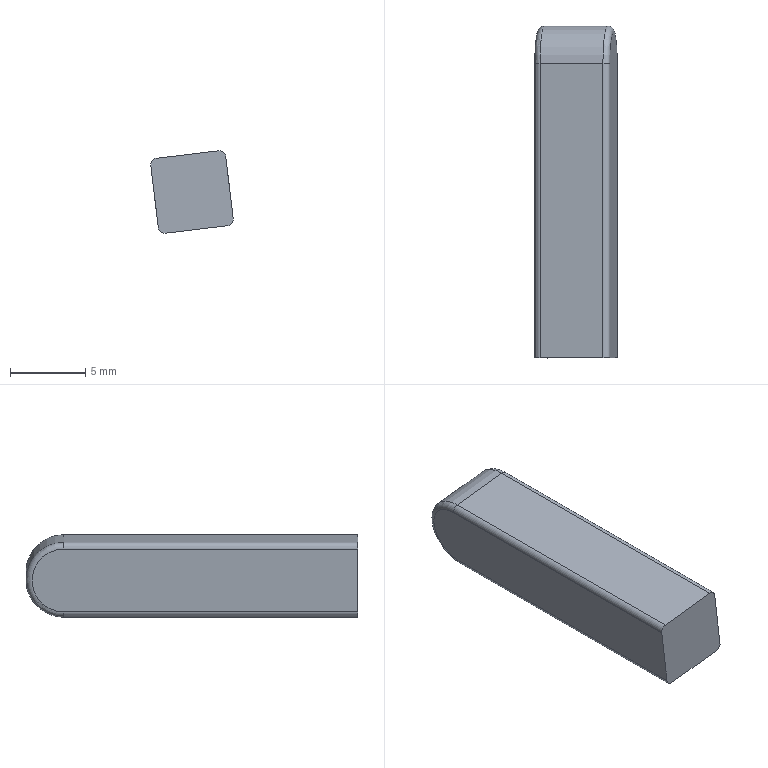Component | SolidWorks | GB_T1096-1979PlainParallelKeyC-type5_25-2 | 1 solid | 13 faces | box 5.47 x 22 x 5.47 mm | volume 533 mm3 | cylinder 6 | plane 5 | torus 2 | commonest cylinder face diameters 0.8 x4 5 x2
STEP:
#1=CARTESIAN_POINT('',(0.06621,2.707,-6.481));
#2=VERTEX_POINT('',#1);
#3=CARTESIAN_POINT('',(0.07799,2.806,-6.578));
#4=VERTEX_POINT('',#3);
#5=CARTESIAN_POINT('',(0.07799,2.707,-6.578));
#6=DIRECTION('',(-0.9928,0.,-0.1196));
#7=DIRECTION('',(0.,-1.,0.));
#8=AXIS2_PLACEMENT_3D('',#5,#6,#7);
#9=CIRCLE('',#8,0.09843);
#10=EDGE_CURVE('',#2,#4,#9,.T.);
#11=ORIENTED_EDGE('',*,*,#10,.T.);
#12=CARTESIAN_POINT('',(-0.08618,2.806,-6.598));
#13=VERTEX_POINT('',#12);
#14=CARTESIAN_POINT('',(0.09362,2.806,-6.577));
#15=DIRECTION('',(-0.9928,0.,-0.1196));
#16=VECTOR('',#15,39.37);
#17=LINE('',#14,#16);
#18=EDGE_CURVE('',#4,#13,#17,.T.);
#19=ORIENTED_EDGE('',*,*,#18,.T.);
#20=CARTESIAN_POINT('',(-0.09796,2.707,-6.501));
#21=VERTEX_POINT('',#20);
#22=CARTESIAN_POINT('',(-0.08618,2.707,-6.598));
#23=DIRECTION('',(0.9928,-0.,0.1196));
#24=DIRECTION('',(0.,-1.,0.));
#25=AXIS2_PLACEMENT_3D('',#22,#23,#24);
#26=CIRCLE('',#25,0.09843);
#27=EDGE_CURVE('',#13,#21,#26,.T.);
#28=ORIENTED_EDGE('',*,*,#27,.T.);
#29=CARTESIAN_POINT('',(0.08184,2.707,-6.479));
#30=DIRECTION('',(-0.9928,0.,-0.1196));
#31=VECTOR('',#30,39.37);
#32=LINE('',#29,#31);
#33=EDGE_CURVE('',#2,#21,#32,.T.);
#34=ORIENTED_EDGE('',*,*,#33,.F.);
#35=EDGE_LOOP('',(#11,#19,#28,#34));
#36=FACE_OUTER_BOUND('',#35,.T.);
#37=CARTESIAN_POINT('',(0.09362,2.707,-6.577));
#38=DIRECTION('',(-0.9928,0.,-0.1196));
#39=DIRECTION('',(0.,1.,0.));
#40=AXIS2_PLACEMENT_3D('',#37,#38,#39);
#41=CYLINDRICAL_SURFACE('',#40,0.09843);
#42=ADVANCED_FACE('',(#36),#41,.T.);
#43=CARTESIAN_POINT('',(0.08373,1.94,-6.495));
#44=VERTEX_POINT('',#43);
#45=CARTESIAN_POINT('',(0.1035,1.94,-6.659));
#46=VERTEX_POINT('',#45);
#47=CARTESIAN_POINT('',(0.1054,1.94,-6.674));
#48=DIRECTION('',(0.1196,0.,-0.9928));
#49=VECTOR('',#48,39.37);
#50=LINE('',#47,#49);
#51=EDGE_CURVE('',#44,#46,#50,.T.);
#52=ORIENTED_EDGE('',*,*,#51,.F.);
#53=CARTESIAN_POINT('',(0.06621,1.94,-6.481));
#54=VERTEX_POINT('',#53);
#55=CARTESIAN_POINT('',(0.06809,1.94,-6.496));
#56=DIRECTION('',(-0.,-1.,-0.));
#57=DIRECTION('',(0.9928,0.,0.1196));
#58=AXIS2_PLACEMENT_3D('',#55,#56,#57);
#59=CIRCLE('',#58,0.01575);
#60=EDGE_CURVE('',#44,#54,#59,.T.);
#61=ORIENTED_EDGE('',*,*,#60,.T.);
#62=CARTESIAN_POINT('',(-0.09796,1.94,-6.501));
#63=VERTEX_POINT('',#62);
#64=CARTESIAN_POINT('',(0.08184,1.94,-6.479));
#65=DIRECTION('',(-0.9928,0.,-0.1196));
#66=VECTOR('',#65,39.37);
#67=LINE('',#64,#66);
#68=EDGE_CURVE('',#54,#63,#67,.T.);
#69=ORIENTED_EDGE('',*,*,#68,.T.);
#70=CARTESIAN_POINT('',(-0.1117,1.94,-6.518));
#71=VERTEX_POINT('',#70);
#72=CARTESIAN_POINT('',(-0.09607,1.94,-6.516));
#73=DIRECTION('',(-0.,-1.,-0.));
#74=DIRECTION('',(0.9928,0.,0.1196));
#75=AXIS2_PLACEMENT_3D('',#72,#73,#74);
#76=CIRCLE('',#75,0.01575);
#77=EDGE_CURVE('',#63,#71,#76,.T.);
#78=ORIENTED_EDGE('',*,*,#77,.T.);
#79=CARTESIAN_POINT('',(-0.09192,1.94,-6.682));
#80=VERTEX_POINT('',#79);
#81=CARTESIAN_POINT('',(-0.09004,1.94,-6.698));
#82=DIRECTION('',(0.1196,0.,-0.9928));
#83=VECTOR('',#82,39.37);
#84=LINE('',#81,#83);
#85=EDGE_CURVE('',#71,#80,#84,.T.);
#86=ORIENTED_EDGE('',*,*,#85,.T.);
#87=CARTESIAN_POINT('',(-0.0744,1.94,-6.696));
#88=VERTEX_POINT('',#87);
#89=CARTESIAN_POINT('',(-0.07629,1.94,-6.68));
#90=DIRECTION('',(-0.,-1.,-0.));
#91=DIRECTION('',(0.9928,0.,0.1196));
#92=AXIS2_PLACEMENT_3D('',#89,#90,#91);
#93=CIRCLE('',#92,0.01575);
#94=EDGE_CURVE('',#80,#88,#93,.T.);
#95=ORIENTED_EDGE('',*,*,#94,.T.);
#96=CARTESIAN_POINT('',(0.08976,1.94,-6.676));
#97=VERTEX_POINT('',#96);
#98=CARTESIAN_POINT('',(0.1054,1.94,-6.674));
#99=DIRECTION('',(-0.9928,0.,-0.1196));
#100=VECTOR('',#99,39.37);
#101=LINE('',#98,#100);
#102=EDGE_CURVE('',#97,#88,#101,.T.);
#103=ORIENTED_EDGE('',*,*,#102,.F.);
#104=CARTESIAN_POINT('',(0.08788,1.94,-6.661));
#105=DIRECTION('',(-0.,-1.,-0.));
#106=DIRECTION('',(0.9928,0.,0.1196));
#107=AXIS2_PLACEMENT_3D('',#104,#105,#106);
#108=CIRCLE('',#107,0.01575);
#109=EDGE_CURVE('',#97,#46,#108,.T.);
#110=ORIENTED_EDGE('',*,*,#109,.T.);
#111=EDGE_LOOP('',(#52,#61,#69,#78,#86,#95,#103,#110));
#112=FACE_OUTER_BOUND('',#111,.T.);
#113=CARTESIAN_POINT('',(0.1054,1.94,-6.674));
#114=DIRECTION('',(0.,1.,0.));
#115=DIRECTION('',(0.9928,-0.,0.1196));
#116=AXIS2_PLACEMENT_3D('',#113,#114,#115);
#117=PLANE('',#116);
#118=ADVANCED_FACE('',(#112),#117,.F.);
#119=CARTESIAN_POINT('',(0.08976,2.707,-6.676));
#120=VERTEX_POINT('',#119);
#121=CARTESIAN_POINT('',(-0.0744,2.707,-6.696));
#122=VERTEX_POINT('',#121);
#123=CARTESIAN_POINT('',(0.1054,2.707,-6.674));
#124=DIRECTION('',(-0.9928,0.,-0.1196));
#125=VECTOR('',#124,39.37);
#126=LINE('',#123,#125);
#127=EDGE_CURVE('',#120,#122,#126,.T.);
#128=ORIENTED_EDGE('',*,*,#127,.F.);
#129=CARTESIAN_POINT('',(0.08976,1.94,-6.676));
#130=DIRECTION('',(-0.,-1.,-0.));
#131=VECTOR('',#130,39.37);
#132=LINE('',#129,#131);
#133=EDGE_CURVE('',#120,#97,#132,.T.);
#134=ORIENTED_EDGE('',*,*,#133,.T.);
#135=ORIENTED_EDGE('',*,*,#102,.T.);
#136=CARTESIAN_POINT('',(-0.0744,2.707,-6.696));
#137=DIRECTION('',(0.,1.,0.));
#138=VECTOR('',#137,39.37);
#139=LINE('',#136,#138);
#140=EDGE_CURVE('',#88,#122,#139,.T.);
#141=ORIENTED_EDGE('',*,*,#140,.T.);
#142=EDGE_LOOP('',(#128,#134,#135,#141));
#143=FACE_OUTER_BOUND('',#142,.T.);
#144=CARTESIAN_POINT('',(0.1054,2.707,-6.674));
#145=DIRECTION('',(-0.1196,-0.,0.9928));
#146=DIRECTION('',(-0.9928,0.,-0.1196));
#147=AXIS2_PLACEMENT_3D('',#144,#145,#146);
#148=PLANE('',#147);
#149=ADVANCED_FACE('',(#143),#148,.F.);
#150=ORIENTED_EDGE('',*,*,#18,.F.);
#151=CARTESIAN_POINT('',(0.07799,2.707,-6.578));
#152=DIRECTION('',(-0.9928,0.,-0.1196));
#153=DIRECTION('',(0.,-1.,0.));
#154=AXIS2_PLACEMENT_3D('',#151,#152,#153);
#155=CIRCLE('',#154,0.09843);
#156=EDGE_CURVE('',#4,#120,#155,.T.);
#157=ORIENTED_EDGE('',*,*,#156,.T.);
#158=ORIENTED_EDGE('',*,*,#127,.T.);
#159=CARTESIAN_POINT('',(-0.08618,2.707,-6.598));
#160=DIRECTION('',(0.9928,-0.,0.1196));
#161=DIRECTION('',(0.,-1.,0.));
#162=AXIS2_PLACEMENT_3D('',#159,#160,#161);
#163=CIRCLE('',#162,0.09843);
#164=EDGE_CURVE('',#122,#13,#163,.T.);
#165=ORIENTED_EDGE('',*,*,#164,.T.);
#166=EDGE_LOOP('',(#150,#157,#158,#165));
#167=FACE_OUTER_BOUND('',#166,.T.);
#168=CARTESIAN_POINT('',(0.09362,2.707,-6.577));
#169=DIRECTION('',(-0.9928,0.,-0.1196));
#170=DIRECTION('',(0.,1.,0.));
#171=AXIS2_PLACEMENT_3D('',#168,#169,#170);
#172=CYLINDRICAL_SURFACE('',#171,0.09843);
#173=ADVANCED_FACE('',(#167),#172,.T.);
#174=ORIENTED_EDGE('',*,*,#68,.F.);
#175=CARTESIAN_POINT('',(0.06621,2.707,-6.481));
#176=DIRECTION('',(0.,1.,0.));
#177=VECTOR('',#176,39.37);
#178=LINE('',#175,#177);
#179=EDGE_CURVE('',#54,#2,#178,.T.);
#180=ORIENTED_EDGE('',*,*,#179,.T.);
#181=ORIENTED_EDGE('',*,*,#33,.T.);
#182=CARTESIAN_POINT('',(-0.09796,2.707,-6.501));
#183=DIRECTION('',(-0.,-1.,-0.));
#184=VECTOR('',#183,39.37);
#185=LINE('',#182,#184);
#186=EDGE_CURVE('',#21,#63,#185,.T.);
#187=ORIENTED_EDGE('',*,*,#186,.T.);
#188=EDGE_LOOP('',(#174,#180,#181,#187));
#189=FACE_OUTER_BOUND('',#188,.T.);
#190=CARTESIAN_POINT('',(0.08184,2.707,-6.479));
#191=DIRECTION('',(0.1196,0.,-0.9928));
#192=DIRECTION('',(0.9928,-0.,0.1196));
#193=AXIS2_PLACEMENT_3D('',#190,#191,#192);
#194=PLANE('',#193);
#195=ADVANCED_FACE('',(#189),#194,.F.);
#196=CARTESIAN_POINT('',(0.1035,2.707,-6.659));
#197=VERTEX_POINT('',#196);
#198=CARTESIAN_POINT('',(0.08373,2.707,-6.495));
#199=VERTEX_POINT('',#198);
#200=CARTESIAN_POINT('',(0.09362,2.707,-6.577));
#201=DIRECTION('',(0.9928,-0.,0.1196));
#202=DIRECTION('',(0.,-1.,0.));
#203=AXIS2_PLACEMENT_3D('',#200,#201,#202);
#204=CIRCLE('',#203,0.08268);
#205=EDGE_CURVE('',#197,#199,#204,.T.);
#206=ORIENTED_EDGE('',*,*,#205,.T.);
#207=CARTESIAN_POINT('',(0.08373,1.94,-6.495));
#208=DIRECTION('',(-0.,-1.,-0.));
#209=VECTOR('',#208,39.37);
#210=LINE('',#207,#209);
#211=EDGE_CURVE('',#199,#44,#210,.T.);
#212=ORIENTED_EDGE('',*,*,#211,.T.);
#213=ORIENTED_EDGE('',*,*,#51,.T.);
#214=CARTESIAN_POINT('',(0.1035,2.707,-6.659));
#215=DIRECTION('',(0.,1.,0.));
#216=VECTOR('',#215,39.37);
#217=LINE('',#214,#216);
#218=EDGE_CURVE('',#46,#197,#217,.T.);
#219=ORIENTED_EDGE('',*,*,#218,.T.);
#220=EDGE_LOOP('',(#206,#212,#213,#219));
#221=FACE_OUTER_BOUND('',#220,.T.);
#222=CARTESIAN_POINT('',(0.09362,2.707,-6.577));
#223=DIRECTION('',(0.9928,-0.,0.1196));
#224=DIRECTION('',(-0.,-1.,-0.));
#225=AXIS2_PLACEMENT_3D('',#222,#223,#224);
#226=PLANE('',#225);
#227=ADVANCED_FACE('',(#221),#226,.T.);
#228=CARTESIAN_POINT('',(-0.1117,2.707,-6.518));
#229=VERTEX_POINT('',#228);
#230=CARTESIAN_POINT('',(-0.09192,2.707,-6.682));
#231=VERTEX_POINT('',#230);
#232=CARTESIAN_POINT('',(-0.1018,2.707,-6.6));
#233=DIRECTION('',(-0.9928,0.,-0.1196));
#234=DIRECTION('',(0.,-1.,0.));
#235=AXIS2_PLACEMENT_3D('',#232,#233,#234);
#236=CIRCLE('',#235,0.08268);
#237=EDGE_CURVE('',#229,#231,#236,.T.);
#238=ORIENTED_EDGE('',*,*,#237,.T.);
#239=CARTESIAN_POINT('',(-0.09192,2.707,-6.682));
#240=DIRECTION('',(-0.,-1.,-0.));
#241=VECTOR('',#240,39.37);
#242=LINE('',#239,#241);
#243=EDGE_CURVE('',#231,#80,#242,.T.);
#244=ORIENTED_EDGE('',*,*,#243,.T.);
#245=ORIENTED_EDGE('',*,*,#85,.F.);
#246=CARTESIAN_POINT('',(-0.1117,2.707,-6.518));
#247=DIRECTION('',(0.,1.,0.));
#248=VECTOR('',#247,39.37);
#249=LINE('',#246,#248);
#250=EDGE_CURVE('',#71,#229,#249,.T.);
#251=ORIENTED_EDGE('',*,*,#250,.T.);
#252=EDGE_LOOP('',(#238,#244,#245,#251));
#253=FACE_OUTER_BOUND('',#252,.T.);
#254=CARTESIAN_POINT('',(-0.1018,2.707,-6.6));
#255=DIRECTION('',(0.9928,-0.,0.1196));
#256=DIRECTION('',(-0.,-1.,-0.));
#257=AXIS2_PLACEMENT_3D('',#254,#255,#256);
#258=PLANE('',#257);
#259=ADVANCED_FACE('',(#253),#258,.F.);
#260=ORIENTED_EDGE('',*,*,#109,.F.);
#261=ORIENTED_EDGE('',*,*,#133,.F.);
#262=CARTESIAN_POINT('',(0.08788,2.707,-6.661));
#263=DIRECTION('',(0.,1.,0.));
#264=DIRECTION('',(0.9928,0.,0.1196));
#265=AXIS2_PLACEMENT_3D('',#262,#263,#264);
#266=CIRCLE('',#265,0.01575);
#267=EDGE_CURVE('',#197,#120,#266,.T.);
#268=ORIENTED_EDGE('',*,*,#267,.F.);
#269=ORIENTED_EDGE('',*,*,#218,.F.);
#270=EDGE_LOOP('',(#260,#261,#268,#269));
#271=FACE_OUTER_BOUND('',#270,.T.);
#272=CARTESIAN_POINT('',(0.08788,2.707,-6.661));
#273=DIRECTION('',(-0.,-1.,-0.));
#274=DIRECTION('',(-0.9928,0.,-0.1196));
#275=AXIS2_PLACEMENT_3D('',#272,#273,#274);
#276=CYLINDRICAL_SURFACE('',#275,0.01575);
#277=ADVANCED_FACE('',(#271),#276,.T.);
#278=ORIENTED_EDGE('',*,*,#267,.T.);
#279=ORIENTED_EDGE('',*,*,#156,.F.);
#280=ORIENTED_EDGE('',*,*,#10,.F.);
#281=CARTESIAN_POINT('',(0.06809,2.707,-6.496));
#282=DIRECTION('',(-0.,-1.,-0.));
#283=DIRECTION('',(-0.9928,0.,-0.1196));
#284=AXIS2_PLACEMENT_3D('',#281,#282,#283);
#285=CIRCLE('',#284,0.01575);
#286=EDGE_CURVE('',#199,#2,#285,.T.);
#287=ORIENTED_EDGE('',*,*,#286,.F.);
#288=ORIENTED_EDGE('',*,*,#205,.F.);
#289=EDGE_LOOP('',(#278,#279,#280,#287,#288));
#290=FACE_OUTER_BOUND('',#289,.T.);
#291=CARTESIAN_POINT('',(0.07799,2.707,-6.578));
#292=DIRECTION('',(0.9928,-0.,0.1196));
#293=DIRECTION('',(-0.,-1.,-0.));
#294=AXIS2_PLACEMENT_3D('',#291,#292,#293);
#295=TOROIDAL_SURFACE('',#294,0.08268,0.01575);
#296=ADVANCED_FACE('',(#290),#295,.T.);
#297=ORIENTED_EDGE('',*,*,#286,.T.);
#298=ORIENTED_EDGE('',*,*,#179,.F.);
#299=ORIENTED_EDGE('',*,*,#60,.F.);
#300=ORIENTED_EDGE('',*,*,#211,.F.);
#301=EDGE_LOOP('',(#297,#298,#299,#300));
#302=FACE_OUTER_BOUND('',#301,.T.);
#303=CARTESIAN_POINT('',(0.06809,2.707,-6.496));
#304=DIRECTION('',(0.,1.,0.));
#305=DIRECTION('',(0.9928,0.,0.1196));
#306=AXIS2_PLACEMENT_3D('',#303,#304,#305);
#307=CYLINDRICAL_SURFACE('',#306,0.01575);
#308=ADVANCED_FACE('',(#302),#307,.T.);
#309=ORIENTED_EDGE('',*,*,#77,.F.);
#310=ORIENTED_EDGE('',*,*,#186,.F.);
#311=CARTESIAN_POINT('',(-0.09607,2.707,-6.516));
#312=DIRECTION('',(0.,1.,0.));
#313=DIRECTION('',(0.9928,0.,0.1196));
#314=AXIS2_PLACEMENT_3D('',#311,#312,#313);
#315=CIRCLE('',#314,0.01575);
#316=EDGE_CURVE('',#229,#21,#315,.T.);
#317=ORIENTED_EDGE('',*,*,#316,.F.);
#318=ORIENTED_EDGE('',*,*,#250,.F.);
#319=EDGE_LOOP('',(#309,#310,#317,#318));
#320=FACE_OUTER_BOUND('',#319,.T.);
#321=CARTESIAN_POINT('',(-0.09607,2.707,-6.516));
#322=DIRECTION('',(-0.,-1.,-0.));
#323=DIRECTION('',(-0.9928,0.,-0.1196));
#324=AXIS2_PLACEMENT_3D('',#321,#322,#323);
#325=CYLINDRICAL_SURFACE('',#324,0.01575);
#326=ADVANCED_FACE('',(#320),#325,.T.);
#327=ORIENTED_EDGE('',*,*,#316,.T.);
#328=ORIENTED_EDGE('',*,*,#27,.F.);
#329=ORIENTED_EDGE('',*,*,#164,.F.);
#330=CARTESIAN_POINT('',(-0.07629,2.707,-6.68));
#331=DIRECTION('',(-0.,-1.,-0.));
#332=DIRECTION('',(-0.9928,0.,-0.1196));
#333=AXIS2_PLACEMENT_3D('',#330,#331,#332);
#334=CIRCLE('',#333,0.01575);
#335=EDGE_CURVE('',#231,#122,#334,.T.);
#336=ORIENTED_EDGE('',*,*,#335,.F.);
#337=ORIENTED_EDGE('',*,*,#237,.F.);
#338=EDGE_LOOP('',(#327,#328,#329,#336,#337));
#339=FACE_OUTER_BOUND('',#338,.T.);
#340=CARTESIAN_POINT('',(-0.08618,2.707,-6.598));
#341=DIRECTION('',(0.9928,-0.,0.1196));
#342=DIRECTION('',(-0.,-1.,-0.));
#343=AXIS2_PLACEMENT_3D('',#340,#341,#342);
#344=TOROIDAL_SURFACE('',#343,0.08268,0.01575);
#345=ADVANCED_FACE('',(#339),#344,.T.);
#346=ORIENTED_EDGE('',*,*,#94,.F.);
#347=ORIENTED_EDGE('',*,*,#243,.F.);
#348=ORIENTED_EDGE('',*,*,#335,.T.);
#349=ORIENTED_EDGE('',*,*,#140,.F.);
#350=EDGE_LOOP('',(#346,#347,#348,#349));
#351=FACE_OUTER_BOUND('',#350,.T.);
#352=CARTESIAN_POINT('',(-0.07629,2.707,-6.68));
#353=DIRECTION('',(0.,1.,0.));
#354=DIRECTION('',(0.9928,0.,0.1196));
#355=AXIS2_PLACEMENT_3D('',#352,#353,#354);
#356=CYLINDRICAL_SURFACE('',#355,0.01575);
#357=ADVANCED_FACE('',(#351),#356,.T.);
#358=CLOSED_SHELL('',(#42,#118,#149,#173,#195,#227,#259,#277,#296,#308,#326,#345,#357));
#359=MANIFOLD_SOLID_BREP('',#358);
#360=CARTESIAN_POINT('',(0.,0.,0.));
#361=DIRECTION('',(0.,0.,1.));
#362=DIRECTION('',(1.,0.,0.));
#363=AXIS2_PLACEMENT_3D('',#360,#361,#362);
#364=(LENGTH_UNIT()NAMED_UNIT(*)SI_UNIT($,.METRE.));
#365=LENGTH_MEASURE_WITH_UNIT(LENGTH_MEASURE(0.0254),#364);
#366=DIMENSIONAL_EXPONENTS(1.,0.,0.,0.,0.,0.,0.);
#367=(CONVERSION_BASED_UNIT('',#365)LENGTH_UNIT()NAMED_UNIT(#366));
#368=UNCERTAINTY_MEASURE_WITH_UNIT(LENGTH_MEASURE(0.00001),#367,'','');
#369=(NAMED_UNIT(*)PLANE_ANGLE_UNIT()SI_UNIT($,.RADIAN.));
#370=(NAMED_UNIT(*)SI_UNIT($,.STERADIAN.)SOLID_ANGLE_UNIT());
#371=(GEOMETRIC_REPRESENTATION_CONTEXT(3)GLOBAL_UNCERTAINTY_ASSIGNED_CONTEXT((#368))GLOBAL_UNIT_ASSIGNED_CONTEXT((#367,#369,#370))REPRESENTATION_CONTEXT('',''));
#372=ADVANCED_BREP_SHAPE_REPRESENTATION('',(#359,#363),#371);
#373=COLOUR_RGB('',0.7922,0.8196,0.9333);
#374=FILL_AREA_STYLE_COLOUR('',#373);
#375=FILL_AREA_STYLE('',(#374));
#376=SURFACE_STYLE_FILL_AREA(#375);
#377=SURFACE_SIDE_STYLE('',(#376));
#378=SURFACE_STYLE_USAGE(.BOTH.,#377);
#379=PRESENTATION_STYLE_ASSIGNMENT((#378));
#380=STYLED_ITEM('',(#379),#359);
#381=PRESENTATION_LAYER_ASSIGNMENT('','',(#380));
#382=(LENGTH_UNIT()NAMED_UNIT(*)SI_UNIT($,.METRE.));
#383=LENGTH_MEASURE_WITH_UNIT(LENGTH_MEASURE(0.0254),#382);
#384=DIMENSIONAL_EXPONENTS(1.,0.,0.,0.,0.,0.,0.);
#385=(CONVERSION_BASED_UNIT('',#383)LENGTH_UNIT()NAMED_UNIT(#384));
#386=UNCERTAINTY_MEASURE_WITH_UNIT(LENGTH_MEASURE(0.00001),#385,'','');
#387=(NAMED_UNIT(*)PLANE_ANGLE_UNIT()SI_UNIT($,.RADIAN.));
#388=(NAMED_UNIT(*)SI_UNIT($,.STERADIAN.)SOLID_ANGLE_UNIT());
#389=(GEOMETRIC_REPRESENTATION_CONTEXT(3)GLOBAL_UNCERTAINTY_ASSIGNED_CONTEXT((#386))GLOBAL_UNIT_ASSIGNED_CONTEXT((#385,#387,#388))REPRESENTATION_CONTEXT('',''));
#390=MECHANICAL_DESIGN_GEOMETRIC_PRESENTATION_REPRESENTATION('',(#380),#389);